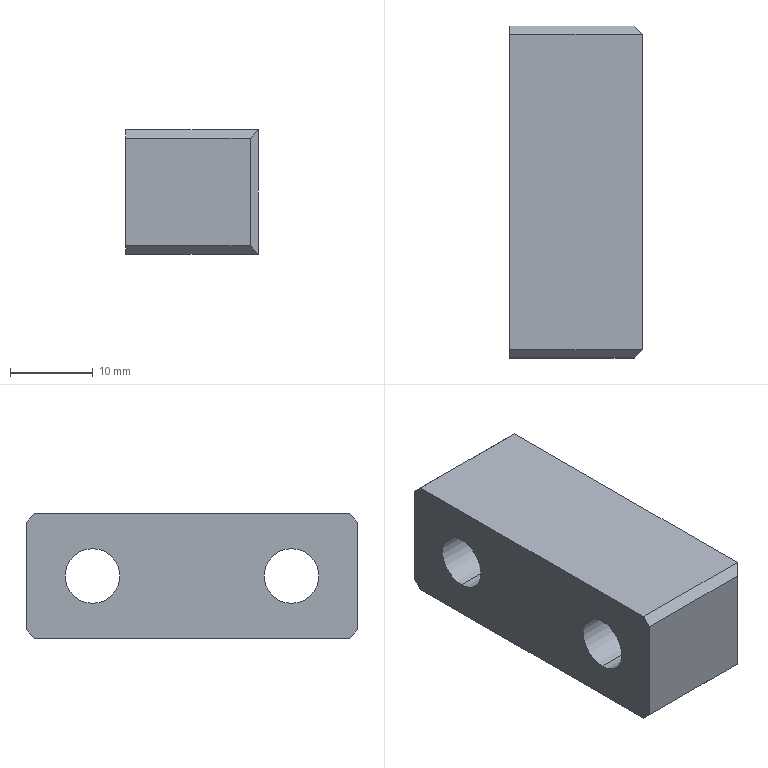Component | SolidWorks | ConveyorScrewAdjustmentSeatOne-2 | 1 solid | 22 faces | box 16 x 40 x 15 mm | volume 7389 mm3 | plane 14 | cylinder 8 | commonest cylinder face diameters 11 x4 6.6 x4 | material Plain Carbon Steel
build123d program:
from build123d import *

# Parameters (mm, degrees)
SKETCH1_W                                            = 15
SKETCH1_H                                            = 40
BOSS_EXTRUDE1_DEPTH                                  = 16
HOLE_SIZE_ACCORDING_TO_TYPE_1_OF_HEXAGON_D           = 6.6
HOLE_SIZE_ACCORDING_TO_TYPE_1_OF_HEXAGON_CBORE_D     = 11
HOLE_SIZE_ACCORDING_TO_TYPE_1_OF_HEXAGON_CBORE_DEPTH = 8.8
CHAMFER1_SIZE                                        = 1


with BuildPart() as part:
    # Sketch1 → Boss-Extrude1 (new body)
    with BuildSketch(Plane(origin=(0, 0, 0), x_dir=(0, 0, -1), z_dir=(1, 0, 0))):
        Rectangle(SKETCH1_W, SKETCH1_H)
    extrude(amount=BOSS_EXTRUDE1_DEPTH)

    # Hole Size according to type 1 of hexagon (through all)
    with Locations(Plane(origin=(16, 0, 0), x_dir=(0, 0, -1), z_dir=(1, 0, 0))):
        with Locations((0, 12), (0, -12)):
            CounterBoreHole(HOLE_SIZE_ACCORDING_TO_TYPE_1_OF_HEXAGON_D / 2, HOLE_SIZE_ACCORDING_TO_TYPE_1_OF_HEXAGON_CBORE_D / 2, HOLE_SIZE_ACCORDING_TO_TYPE_1_OF_HEXAGON_CBORE_DEPTH)

    # Chamfer1
    chamfer1_edges = [part.edges().sort_by_distance(p)[0] for p in [
        (16, -20, 0),
        (16, 20, 0),
        (8, -20, -7.5),
        (8, -20, 7.5),
        (8, 20, 7.5),
        (8, 20, -7.5),
    ]]
    chamfer(chamfer1_edges, length=CHAMFER1_SIZE)


solid = part.part

# Placed as in the assembly
solid = solid.moved(Location((47.45, 5.646, 227.5), (0, 0, 0)))
STEP:
#1=COLOUR_RGB('',0.7922,0.8196,0.9333);
#2=FILL_AREA_STYLE_COLOUR('',#1);
#3=FILL_AREA_STYLE('',(#2));
#4=SURFACE_STYLE_FILL_AREA(#3);
#5=SURFACE_SIDE_STYLE('',(#4));
#6=SURFACE_STYLE_USAGE(.BOTH.,#5);
#7=PRESENTATION_STYLE_ASSIGNMENT((#6));
#8=CARTESIAN_POINT('',(2.152,0.6947,9.173));
#9=VERTEX_POINT('',#8);
#10=CARTESIAN_POINT('',(2.152,0.6947,8.74));
#11=VERTEX_POINT('',#10);
#12=CARTESIAN_POINT('',(2.152,0.6947,8.957));
#13=DIRECTION('',(1.,0.,0.));
#14=DIRECTION('',(0.,0.,-1.));
#15=AXIS2_PLACEMENT_3D('',#12,#13,#14);
#16=CIRCLE('',#15,0.2165);
#17=EDGE_CURVE('',#9,#11,#16,.T.);
#18=ORIENTED_EDGE('',*,*,#17,.F.);
#19=CARTESIAN_POINT('',(2.498,0.6947,9.173));
#20=VERTEX_POINT('',#19);
#21=CARTESIAN_POINT('',(2.498,0.6947,9.173));
#22=DIRECTION('',(1.,0.,0.));
#23=VECTOR('',#22,39.37);
#24=LINE('',#21,#23);
#25=EDGE_CURVE('',#9,#20,#24,.T.);
#26=ORIENTED_EDGE('',*,*,#25,.T.);
#27=CARTESIAN_POINT('',(2.498,0.6947,8.74));
#28=VERTEX_POINT('',#27);
#29=CARTESIAN_POINT('',(2.498,0.6947,8.957));
#30=DIRECTION('',(1.,0.,0.));
#31=DIRECTION('',(0.,0.,-1.));
#32=AXIS2_PLACEMENT_3D('',#29,#30,#31);
#33=CIRCLE('',#32,0.2165);
#34=EDGE_CURVE('',#20,#28,#33,.T.);
#35=ORIENTED_EDGE('',*,*,#34,.T.);
#36=CARTESIAN_POINT('',(2.498,0.6947,8.74));
#37=DIRECTION('',(1.,0.,0.));
#38=VECTOR('',#37,39.37);
#39=LINE('',#36,#38);
#40=EDGE_CURVE('',#11,#28,#39,.T.);
#41=ORIENTED_EDGE('',*,*,#40,.F.);
#42=EDGE_LOOP('',(#18,#26,#35,#41));
#43=FACE_OUTER_BOUND('',#42,.T.);
#44=CARTESIAN_POINT('',(2.498,0.6947,8.957));
#45=DIRECTION('',(1.,0.,0.));
#46=DIRECTION('',(0.,0.,-1.));
#47=AXIS2_PLACEMENT_3D('',#44,#45,#46);
#48=CYLINDRICAL_SURFACE('',#47,0.2165);
#49=ADVANCED_FACE('',(#43),#48,.F.);
#50=CARTESIAN_POINT('',(1.868,0.6947,9.087));
#51=VERTEX_POINT('',#50);
#52=CARTESIAN_POINT('',(1.868,0.6947,8.827));
#53=VERTEX_POINT('',#52);
#54=CARTESIAN_POINT('',(1.868,0.6947,8.957));
#55=DIRECTION('',(1.,0.,0.));
#56=DIRECTION('',(0.,0.,-1.));
#57=AXIS2_PLACEMENT_3D('',#54,#55,#56);
#58=CIRCLE('',#57,0.1299);
#59=EDGE_CURVE('',#51,#53,#58,.T.);
#60=ORIENTED_EDGE('',*,*,#59,.F.);
#61=CARTESIAN_POINT('',(2.152,0.6947,9.087));
#62=VERTEX_POINT('',#61);
#63=CARTESIAN_POINT('',(2.498,0.6947,9.087));
#64=DIRECTION('',(1.,0.,0.));
#65=VECTOR('',#64,39.37);
#66=LINE('',#63,#65);
#67=EDGE_CURVE('',#51,#62,#66,.T.);
#68=ORIENTED_EDGE('',*,*,#67,.T.);
#69=CARTESIAN_POINT('',(2.152,0.6947,8.827));
#70=VERTEX_POINT('',#69);
#71=CARTESIAN_POINT('',(2.152,0.6947,8.957));
#72=DIRECTION('',(1.,0.,0.));
#73=DIRECTION('',(0.,0.,-1.));
#74=AXIS2_PLACEMENT_3D('',#71,#72,#73);
#75=CIRCLE('',#74,0.1299);
#76=EDGE_CURVE('',#62,#70,#75,.T.);
#77=ORIENTED_EDGE('',*,*,#76,.T.);
#78=CARTESIAN_POINT('',(2.498,0.6947,8.827));
#79=DIRECTION('',(1.,0.,0.));
#80=VECTOR('',#79,39.37);
#81=LINE('',#78,#80);
#82=EDGE_CURVE('',#53,#70,#81,.T.);
#83=ORIENTED_EDGE('',*,*,#82,.F.);
#84=EDGE_LOOP('',(#60,#68,#77,#83));
#85=FACE_OUTER_BOUND('',#84,.T.);
#86=CARTESIAN_POINT('',(2.498,0.6947,8.957));
#87=DIRECTION('',(1.,0.,0.));
#88=DIRECTION('',(0.,0.,-1.));
#89=AXIS2_PLACEMENT_3D('',#86,#87,#88);
#90=CYLINDRICAL_SURFACE('',#89,0.1299);
#91=ADVANCED_FACE('',(#85),#90,.F.);
#92=CARTESIAN_POINT('',(2.152,-0.2502,9.173));
#93=VERTEX_POINT('',#92);
#94=CARTESIAN_POINT('',(2.152,-0.2502,8.74));
#95=VERTEX_POINT('',#94);
#96=CARTESIAN_POINT('',(2.152,-0.2502,8.957));
#97=DIRECTION('',(1.,0.,0.));
#98=DIRECTION('',(0.,0.,-1.));
#99=AXIS2_PLACEMENT_3D('',#96,#97,#98);
#100=CIRCLE('',#99,0.2165);
#101=EDGE_CURVE('',#93,#95,#100,.T.);
#102=ORIENTED_EDGE('',*,*,#101,.F.);
#103=CARTESIAN_POINT('',(2.498,-0.2502,9.173));
#104=VERTEX_POINT('',#103);
#105=CARTESIAN_POINT('',(2.498,-0.2502,9.173));
#106=DIRECTION('',(1.,0.,0.));
#107=VECTOR('',#106,39.37);
#108=LINE('',#105,#107);
#109=EDGE_CURVE('',#93,#104,#108,.T.);
#110=ORIENTED_EDGE('',*,*,#109,.T.);
#111=CARTESIAN_POINT('',(2.498,-0.2502,8.74));
#112=VERTEX_POINT('',#111);
#113=CARTESIAN_POINT('',(2.498,-0.2502,8.957));
#114=DIRECTION('',(1.,0.,0.));
#115=DIRECTION('',(0.,0.,-1.));
#116=AXIS2_PLACEMENT_3D('',#113,#114,#115);
#117=CIRCLE('',#116,0.2165);
#118=EDGE_CURVE('',#104,#112,#117,.T.);
#119=ORIENTED_EDGE('',*,*,#118,.T.);
#120=CARTESIAN_POINT('',(2.498,-0.2502,8.74));
#121=DIRECTION('',(1.,0.,0.));
#122=VECTOR('',#121,39.37);
#123=LINE('',#120,#122);
#124=EDGE_CURVE('',#95,#112,#123,.T.);
#125=ORIENTED_EDGE('',*,*,#124,.F.);
#126=EDGE_LOOP('',(#102,#110,#119,#125));
#127=FACE_OUTER_BOUND('',#126,.T.);
#128=CARTESIAN_POINT('',(2.498,-0.2502,8.957));
#129=DIRECTION('',(1.,0.,0.));
#130=DIRECTION('',(0.,0.,-1.));
#131=AXIS2_PLACEMENT_3D('',#128,#129,#130);
#132=CYLINDRICAL_SURFACE('',#131,0.2165);
#133=ADVANCED_FACE('',(#127),#132,.F.);
#134=CARTESIAN_POINT('',(1.868,-0.2502,9.087));
#135=VERTEX_POINT('',#134);
#136=CARTESIAN_POINT('',(1.868,-0.2502,8.827));
#137=VERTEX_POINT('',#136);
#138=CARTESIAN_POINT('',(1.868,-0.2502,8.957));
#139=DIRECTION('',(1.,0.,0.));
#140=DIRECTION('',(0.,0.,-1.));
#141=AXIS2_PLACEMENT_3D('',#138,#139,#140);
#142=CIRCLE('',#141,0.1299);
#143=EDGE_CURVE('',#135,#137,#142,.T.);
#144=ORIENTED_EDGE('',*,*,#143,.F.);
#145=CARTESIAN_POINT('',(2.152,-0.2502,9.087));
#146=VERTEX_POINT('',#145);
#147=CARTESIAN_POINT('',(2.498,-0.2502,9.087));
#148=DIRECTION('',(1.,0.,0.));
#149=VECTOR('',#148,39.37);
#150=LINE('',#147,#149);
#151=EDGE_CURVE('',#135,#146,#150,.T.);
#152=ORIENTED_EDGE('',*,*,#151,.T.);
#153=CARTESIAN_POINT('',(2.152,-0.2502,8.827));
#154=VERTEX_POINT('',#153);
#155=CARTESIAN_POINT('',(2.152,-0.2502,8.957));
#156=DIRECTION('',(1.,0.,0.));
#157=DIRECTION('',(0.,0.,-1.));
#158=AXIS2_PLACEMENT_3D('',#155,#156,#157);
#159=CIRCLE('',#158,0.1299);
#160=EDGE_CURVE('',#146,#154,#159,.T.);
#161=ORIENTED_EDGE('',*,*,#160,.T.);
#162=CARTESIAN_POINT('',(2.498,-0.2502,8.827));
#163=DIRECTION('',(1.,0.,0.));
#164=VECTOR('',#163,39.37);
#165=LINE('',#162,#164);
#166=EDGE_CURVE('',#137,#154,#165,.T.);
#167=ORIENTED_EDGE('',*,*,#166,.F.);
#168=EDGE_LOOP('',(#144,#152,#161,#167));
#169=FACE_OUTER_BOUND('',#168,.T.);
#170=CARTESIAN_POINT('',(2.498,-0.2502,8.957));
#171=DIRECTION('',(1.,0.,0.));
#172=DIRECTION('',(0.,0.,-1.));
#173=AXIS2_PLACEMENT_3D('',#170,#171,#172);
#174=CYLINDRICAL_SURFACE('',#173,0.1299);
#175=ADVANCED_FACE('',(#169),#174,.F.);
#176=CARTESIAN_POINT('',(2.498,-0.5258,8.661));
#177=VERTEX_POINT('',#176);
#178=CARTESIAN_POINT('',(2.498,0.9703,8.661));
#179=VERTEX_POINT('',#178);
#180=CARTESIAN_POINT('',(2.498,-0.5651,8.661));
#181=DIRECTION('',(0.,1.,0.));
#182=VECTOR('',#181,39.37);
#183=LINE('',#180,#182);
#184=EDGE_CURVE('',#177,#179,#183,.T.);
#185=ORIENTED_EDGE('',*,*,#184,.F.);
#186=CARTESIAN_POINT('',(1.868,-0.5258,8.661));
#187=VERTEX_POINT('',#186);
#188=CARTESIAN_POINT('',(2.498,-0.5258,8.661));
#189=DIRECTION('',(-1.,0.,0.));
#190=VECTOR('',#189,39.37);
#191=LINE('',#188,#190);
#192=EDGE_CURVE('',#177,#187,#191,.T.);
#193=ORIENTED_EDGE('',*,*,#192,.T.);
#194=CARTESIAN_POINT('',(1.868,0.9703,8.661));
#195=VERTEX_POINT('',#194);
#196=CARTESIAN_POINT('',(1.868,-0.5651,8.661));
#197=DIRECTION('',(0.,1.,0.));
#198=VECTOR('',#197,39.37);
#199=LINE('',#196,#198);
#200=EDGE_CURVE('',#187,#195,#199,.T.);
#201=ORIENTED_EDGE('',*,*,#200,.T.);
#202=CARTESIAN_POINT('',(2.498,0.9703,8.661));
#203=DIRECTION('',(1.,0.,0.));
#204=VECTOR('',#203,39.37);
#205=LINE('',#202,#204);
#206=EDGE_CURVE('',#195,#179,#205,.T.);
#207=ORIENTED_EDGE('',*,*,#206,.T.);
#208=EDGE_LOOP('',(#185,#193,#201,#207));
#209=FACE_OUTER_BOUND('',#208,.T.);
#210=CARTESIAN_POINT('',(2.498,-0.5651,8.661));
#211=DIRECTION('',(0.,0.,1.));
#212=DIRECTION('',(1.,0.,0.));
#213=AXIS2_PLACEMENT_3D('',#210,#211,#212);
#214=PLANE('',#213);
#215=ADVANCED_FACE('',(#209),#214,.F.);
#216=CARTESIAN_POINT('',(1.868,1.01,8.701));
#217=VERTEX_POINT('',#216);
#218=CARTESIAN_POINT('',(1.868,1.01,9.213));
#219=VERTEX_POINT('',#218);
#220=CARTESIAN_POINT('',(1.868,1.01,9.252));
#221=DIRECTION('',(0.,0.,1.));
#222=VECTOR('',#221,39.37);
#223=LINE('',#220,#222);
#224=EDGE_CURVE('',#217,#219,#223,.T.);
#225=ORIENTED_EDGE('',*,*,#224,.T.);
#226=CARTESIAN_POINT('',(2.459,1.01,9.213));
#227=VERTEX_POINT('',#226);
#228=CARTESIAN_POINT('',(2.498,1.01,9.213));
#229=DIRECTION('',(1.,0.,0.));
#230=VECTOR('',#229,39.37);
#231=LINE('',#228,#230);
#232=EDGE_CURVE('',#219,#227,#231,.T.);
#233=ORIENTED_EDGE('',*,*,#232,.T.);
#234=CARTESIAN_POINT('',(2.459,1.01,8.701));
#235=VERTEX_POINT('',#234);
#236=CARTESIAN_POINT('',(2.459,1.01,9.252));
#237=DIRECTION('',(0.,0.,-1.));
#238=VECTOR('',#237,39.37);
#239=LINE('',#236,#238);
#240=EDGE_CURVE('',#227,#235,#239,.T.);
#241=ORIENTED_EDGE('',*,*,#240,.T.);
#242=CARTESIAN_POINT('',(2.498,1.01,8.701));
#243=DIRECTION('',(-1.,0.,0.));
#244=VECTOR('',#243,39.37);
#245=LINE('',#242,#244);
#246=EDGE_CURVE('',#235,#217,#245,.T.);
#247=ORIENTED_EDGE('',*,*,#246,.T.);
#248=EDGE_LOOP('',(#225,#233,#241,#247));
#249=FACE_OUTER_BOUND('',#248,.T.);
#250=CARTESIAN_POINT('',(2.498,1.01,9.252));
#251=DIRECTION('',(0.,-1.,0.));
#252=DIRECTION('',(0.,0.,-1.));
#253=AXIS2_PLACEMENT_3D('',#250,#251,#252);
#254=PLANE('',#253);
#255=ADVANCED_FACE('',(#249),#254,.F.);
#256=CARTESIAN_POINT('',(1.868,0.9703,9.252));
#257=VERTEX_POINT('',#256);
#258=CARTESIAN_POINT('',(1.868,-0.5258,9.252));
#259=VERTEX_POINT('',#258);
#260=CARTESIAN_POINT('',(1.868,-0.5651,9.252));
#261=DIRECTION('',(0.,-1.,0.));
#262=VECTOR('',#261,39.37);
#263=LINE('',#260,#262);
#264=EDGE_CURVE('',#257,#259,#263,.T.);
#265=ORIENTED_EDGE('',*,*,#264,.T.);
#266=CARTESIAN_POINT('',(2.498,-0.5258,9.252));
#267=VERTEX_POINT('',#266);
#268=CARTESIAN_POINT('',(2.498,-0.5258,9.252));
#269=DIRECTION('',(1.,0.,0.));
#270=VECTOR('',#269,39.37);
#271=LINE('',#268,#270);
#272=EDGE_CURVE('',#259,#267,#271,.T.);
#273=ORIENTED_EDGE('',*,*,#272,.T.);
#274=CARTESIAN_POINT('',(2.498,0.9703,9.252));
#275=VERTEX_POINT('',#274);
#276=CARTESIAN_POINT('',(2.498,-0.5651,9.252));
#277=DIRECTION('',(0.,-1.,0.));
#278=VECTOR('',#277,39.37);
#279=LINE('',#276,#278);
#280=EDGE_CURVE('',#275,#267,#279,.T.);
#281=ORIENTED_EDGE('',*,*,#280,.F.);
#282=CARTESIAN_POINT('',(2.498,0.9703,9.252));
#283=DIRECTION('',(-1.,0.,0.));
#284=VECTOR('',#283,39.37);
#285=LINE('',#282,#284);
#286=EDGE_CURVE('',#275,#257,#285,.T.);
#287=ORIENTED_EDGE('',*,*,#286,.T.);
#288=EDGE_LOOP('',(#265,#273,#281,#287));
#289=FACE_OUTER_BOUND('',#288,.T.);
#290=CARTESIAN_POINT('',(2.498,-0.5651,9.252));
#291=DIRECTION('',(0.,0.,-1.));
#292=DIRECTION('',(-1.,0.,0.));
#293=AXIS2_PLACEMENT_3D('',#290,#291,#292);
#294=PLANE('',#293);
#295=ADVANCED_FACE('',(#289),#294,.F.);
#296=CARTESIAN_POINT('',(1.868,-0.5651,9.213));
#297=VERTEX_POINT('',#296);
#298=CARTESIAN_POINT('',(1.868,-0.5651,8.701));
#299=VERTEX_POINT('',#298);
#300=CARTESIAN_POINT('',(1.868,-0.5651,9.252));
#301=DIRECTION('',(0.,0.,-1.));
#302=VECTOR('',#301,39.37);
#303=LINE('',#300,#302);
#304=EDGE_CURVE('',#297,#299,#303,.T.);
#305=ORIENTED_EDGE('',*,*,#304,.T.);
#306=CARTESIAN_POINT('',(2.459,-0.5651,8.701));
#307=VERTEX_POINT('',#306);
#308=CARTESIAN_POINT('',(2.498,-0.5651,8.701));
#309=DIRECTION('',(1.,0.,0.));
#310=VECTOR('',#309,39.37);
#311=LINE('',#308,#310);
#312=EDGE_CURVE('',#299,#307,#311,.T.);
#313=ORIENTED_EDGE('',*,*,#312,.T.);
#314=CARTESIAN_POINT('',(2.459,-0.5651,9.213));
#315=VERTEX_POINT('',#314);
#316=CARTESIAN_POINT('',(2.459,-0.5651,9.252));
#317=DIRECTION('',(0.,0.,1.));
#318=VECTOR('',#317,39.37);
#319=LINE('',#316,#318);
#320=EDGE_CURVE('',#307,#315,#319,.T.);
#321=ORIENTED_EDGE('',*,*,#320,.T.);
#322=CARTESIAN_POINT('',(2.498,-0.5651,9.213));
#323=DIRECTION('',(-1.,0.,0.));
#324=VECTOR('',#323,39.37);
#325=LINE('',#322,#324);
#326=EDGE_CURVE('',#315,#297,#325,.T.);
#327=ORIENTED_EDGE('',*,*,#326,.T.);
#328=EDGE_LOOP('',(#305,#313,#321,#327));
#329=FACE_OUTER_BOUND('',#328,.T.);
#330=CARTESIAN_POINT('',(2.498,-0.5651,9.252));
#331=DIRECTION('',(0.,1.,0.));
#332=DIRECTION('',(0.,0.,1.));
#333=AXIS2_PLACEMENT_3D('',#330,#331,#332);
#334=PLANE('',#333);
#335=ADVANCED_FACE('',(#329),#334,.F.);
#336=CARTESIAN_POINT('',(2.498,0.6947,8.957));
#337=DIRECTION('',(1.,0.,0.));
#338=DIRECTION('',(0.,0.,-1.));
#339=AXIS2_PLACEMENT_3D('',#336,#337,#338);
#340=CIRCLE('',#339,0.2165);
#341=EDGE_CURVE('',#28,#20,#340,.T.);
#342=ORIENTED_EDGE('',*,*,#341,.F.);
#343=ORIENTED_EDGE('',*,*,#34,.F.);
#344=EDGE_LOOP('',(#342,#343));
#345=FACE_BOUND('',#344,.T.);
#346=CARTESIAN_POINT('',(2.498,-0.2502,8.957));
#347=DIRECTION('',(1.,0.,0.));
#348=DIRECTION('',(0.,0.,-1.));
#349=AXIS2_PLACEMENT_3D('',#346,#347,#348);
#350=CIRCLE('',#349,0.2165);
#351=EDGE_CURVE('',#112,#104,#350,.T.);
#352=ORIENTED_EDGE('',*,*,#351,.F.);
#353=ORIENTED_EDGE('',*,*,#118,.F.);
#354=EDGE_LOOP('',(#352,#353));
#355=FACE_BOUND('',#354,.T.);
#356=ORIENTED_EDGE('',*,*,#280,.T.);
#357=CARTESIAN_POINT('',(2.498,-0.5258,8.957));
#358=DIRECTION('',(0.,0.,-1.));
#359=VECTOR('',#358,39.37);
#360=LINE('',#357,#359);
#361=EDGE_CURVE('',#267,#177,#360,.T.);
#362=ORIENTED_EDGE('',*,*,#361,.T.);
#363=ORIENTED_EDGE('',*,*,#184,.T.);
#364=CARTESIAN_POINT('',(2.498,0.9703,8.957));
#365=DIRECTION('',(0.,0.,1.));
#366=VECTOR('',#365,39.37);
#367=LINE('',#364,#366);
#368=EDGE_CURVE('',#179,#275,#367,.T.);
#369=ORIENTED_EDGE('',*,*,#368,.T.);
#370=EDGE_LOOP('',(#356,#362,#363,#369));
#371=FACE_OUTER_BOUND('',#370,.T.);
#372=CARTESIAN_POINT('',(2.498,0.2223,8.957));
#373=DIRECTION('',(-1.,0.,0.));
#374=DIRECTION('',(0.,0.,1.));
#375=AXIS2_PLACEMENT_3D('',#372,#373,#374);
#376=PLANE('',#375);
#377=ADVANCED_FACE('',(#345,#355,#371),#376,.F.);
#378=CARTESIAN_POINT('',(1.868,0.6947,8.957));
#379=DIRECTION('',(1.,0.,0.));
#380=DIRECTION('',(0.,0.,-1.));
#381=AXIS2_PLACEMENT_3D('',#378,#379,#380);
#382=CIRCLE('',#381,0.1299);
#383=EDGE_CURVE('',#53,#51,#382,.T.);
#384=ORIENTED_EDGE('',*,*,#383,.T.);
#385=ORIENTED_EDGE('',*,*,#59,.T.);
#386=EDGE_LOOP('',(#384,#385));
#387=FACE_BOUND('',#386,.T.);
#388=CARTESIAN_POINT('',(1.868,-0.2502,8.957));
#389=DIRECTION('',(1.,0.,0.));
#390=DIRECTION('',(0.,0.,-1.));
#391=AXIS2_PLACEMENT_3D('',#388,#389,#390);
#392=CIRCLE('',#391,0.1299);
#393=EDGE_CURVE('',#137,#135,#392,.T.);
#394=ORIENTED_EDGE('',*,*,#393,.T.);
#395=ORIENTED_EDGE('',*,*,#143,.T.);
#396=EDGE_LOOP('',(#394,#395));
#397=FACE_BOUND('',#396,.T.);
#398=ORIENTED_EDGE('',*,*,#200,.F.);
#399=CARTESIAN_POINT('',(1.868,-0.2994,8.435));
#400=DIRECTION('',(0.,-0.7071,0.7071));
#401=VECTOR('',#400,39.37);
#402=LINE('',#399,#401);
#403=EDGE_CURVE('',#187,#299,#402,.T.);
#404=ORIENTED_EDGE('',*,*,#403,.T.);
#405=ORIENTED_EDGE('',*,*,#304,.F.);
#406=CARTESIAN_POINT('',(1.868,-0.2994,9.478));
#407=DIRECTION('',(0.,0.7071,0.7071));
#408=VECTOR('',#407,39.37);
#409=LINE('',#406,#408);
#410=EDGE_CURVE('',#297,#259,#409,.T.);
#411=ORIENTED_EDGE('',*,*,#410,.T.);
#412=ORIENTED_EDGE('',*,*,#264,.F.);
#413=CARTESIAN_POINT('',(1.868,0.7439,9.478));
#414=DIRECTION('',(0.,0.7071,-0.7071));
#415=VECTOR('',#414,39.37);
#416=LINE('',#413,#415);
#417=EDGE_CURVE('',#257,#219,#416,.T.);
#418=ORIENTED_EDGE('',*,*,#417,.T.);
#419=ORIENTED_EDGE('',*,*,#224,.F.);
#420=CARTESIAN_POINT('',(1.868,0.7439,8.435));
#421=DIRECTION('',(0.,-0.7071,-0.7071));
#422=VECTOR('',#421,39.37);
#423=LINE('',#420,#422);
#424=EDGE_CURVE('',#217,#195,#423,.T.);
#425=ORIENTED_EDGE('',*,*,#424,.T.);
#426=EDGE_LOOP('',(#398,#404,#405,#411,#412,#418,#419,#425));
#427=FACE_OUTER_BOUND('',#426,.T.);
#428=CARTESIAN_POINT('',(1.868,0.2223,8.957));
#429=DIRECTION('',(-1.,0.,0.));
#430=DIRECTION('',(0.,0.,1.));
#431=AXIS2_PLACEMENT_3D('',#428,#429,#430);
#432=PLANE('',#431);
#433=ADVANCED_FACE('',(#387,#397,#427),#432,.T.);
#434=ORIENTED_EDGE('',*,*,#151,.F.);
#435=ORIENTED_EDGE('',*,*,#393,.F.);
#436=ORIENTED_EDGE('',*,*,#166,.T.);
#437=CARTESIAN_POINT('',(2.152,-0.2502,8.957));
#438=DIRECTION('',(1.,0.,0.));
#439=DIRECTION('',(0.,0.,-1.));
#440=AXIS2_PLACEMENT_3D('',#437,#438,#439);
#441=CIRCLE('',#440,0.1299);
#442=EDGE_CURVE('',#154,#146,#441,.T.);
#443=ORIENTED_EDGE('',*,*,#442,.T.);
#444=EDGE_LOOP('',(#434,#435,#436,#443));
#445=FACE_OUTER_BOUND('',#444,.T.);
#446=CARTESIAN_POINT('',(2.498,-0.2502,8.957));
#447=DIRECTION('',(1.,0.,0.));
#448=DIRECTION('',(0.,0.,-1.));
#449=AXIS2_PLACEMENT_3D('',#446,#447,#448);
#450=CYLINDRICAL_SURFACE('',#449,0.1299);
#451=ADVANCED_FACE('',(#445),#450,.F.);
#452=ORIENTED_EDGE('',*,*,#442,.F.);
#453=ORIENTED_EDGE('',*,*,#160,.F.);
#454=EDGE_LOOP('',(#452,#453));
#455=FACE_BOUND('',#454,.T.);
#456=CARTESIAN_POINT('',(2.152,-0.2502,8.957));
#457=DIRECTION('',(1.,0.,0.));
#458=DIRECTION('',(0.,0.,-1.));
#459=AXIS2_PLACEMENT_3D('',#456,#457,#458);
#460=CIRCLE('',#459,0.2165);
#461=EDGE_CURVE('',#95,#93,#460,.T.);
#462=ORIENTED_EDGE('',*,*,#461,.T.);
#463=ORIENTED_EDGE('',*,*,#101,.T.);
#464=EDGE_LOOP('',(#462,#463));
#465=FACE_OUTER_BOUND('',#464,.T.);
#466=CARTESIAN_POINT('',(2.152,-0.1202,8.957));
#467=DIRECTION('',(-1.,0.,0.));
#468=DIRECTION('',(0.,0.,1.));
#469=AXIS2_PLACEMENT_3D('',#466,#467,#468);
#470=PLANE('',#469);
#471=ADVANCED_FACE('',(#455,#465),#470,.F.);
#472=ORIENTED_EDGE('',*,*,#109,.F.);
#473=ORIENTED_EDGE('',*,*,#461,.F.);
#474=ORIENTED_EDGE('',*,*,#124,.T.);
#475=ORIENTED_EDGE('',*,*,#351,.T.);
#476=EDGE_LOOP('',(#472,#473,#474,#475));
#477=FACE_OUTER_BOUND('',#476,.T.);
#478=CARTESIAN_POINT('',(2.498,-0.2502,8.957));
#479=DIRECTION('',(1.,0.,0.));
#480=DIRECTION('',(0.,0.,-1.));
#481=AXIS2_PLACEMENT_3D('',#478,#479,#480);
#482=CYLINDRICAL_SURFACE('',#481,0.2165);
#483=ADVANCED_FACE('',(#477),#482,.F.);
#484=ORIENTED_EDGE('',*,*,#67,.F.);
#485=ORIENTED_EDGE('',*,*,#383,.F.);
#486=ORIENTED_EDGE('',*,*,#82,.T.);
#487=CARTESIAN_POINT('',(2.152,0.6947,8.957));
#488=DIRECTION('',(1.,0.,0.));
#489=DIRECTION('',(0.,0.,-1.));
#490=AXIS2_PLACEMENT_3D('',#487,#488,#489);
#491=CIRCLE('',#490,0.1299);
#492=EDGE_CURVE('',#70,#62,#491,.T.);
#493=ORIENTED_EDGE('',*,*,#492,.T.);
#494=EDGE_LOOP('',(#484,#485,#486,#493));
#495=FACE_OUTER_BOUND('',#494,.T.);
#496=CARTESIAN_POINT('',(2.498,0.6947,8.957));
#497=DIRECTION('',(1.,0.,0.));
#498=DIRECTION('',(0.,0.,-1.));
#499=AXIS2_PLACEMENT_3D('',#496,#497,#498);
#500=CYLINDRICAL_SURFACE('',#499,0.1299);
#501=ADVANCED_FACE('',(#495),#500,.F.);
#502=ORIENTED_EDGE('',*,*,#492,.F.);
#503=ORIENTED_EDGE('',*,*,#76,.F.);
#504=EDGE_LOOP('',(#502,#503));
#505=FACE_BOUND('',#504,.T.);
#506=CARTESIAN_POINT('',(2.152,0.6947,8.957));
#507=DIRECTION('',(1.,0.,0.));
#508=DIRECTION('',(0.,0.,-1.));
#509=AXIS2_PLACEMENT_3D('',#506,#507,#508);
#510=CIRCLE('',#509,0.2165);
#511=EDGE_CURVE('',#11,#9,#510,.T.);
#512=ORIENTED_EDGE('',*,*,#511,.T.);
#513=ORIENTED_EDGE('',*,*,#17,.T.);
#514=EDGE_LOOP('',(#512,#513));
#515=FACE_OUTER_BOUND('',#514,.T.);
#516=CARTESIAN_POINT('',(2.152,0.8246,8.957));
#517=DIRECTION('',(-1.,0.,0.));
#518=DIRECTION('',(0.,0.,1.));
#519=AXIS2_PLACEMENT_3D('',#516,#517,#518);
#520=PLANE('',#519);
#521=ADVANCED_FACE('',(#505,#515),#520,.F.);
#522=ORIENTED_EDGE('',*,*,#25,.F.);
#523=ORIENTED_EDGE('',*,*,#511,.F.);
#524=ORIENTED_EDGE('',*,*,#40,.T.);
#525=ORIENTED_EDGE('',*,*,#341,.T.);
#526=EDGE_LOOP('',(#522,#523,#524,#525));
#527=FACE_OUTER_BOUND('',#526,.T.);
#528=CARTESIAN_POINT('',(2.498,0.6947,8.957));
#529=DIRECTION('',(1.,0.,0.));
#530=DIRECTION('',(0.,0.,-1.));
#531=AXIS2_PLACEMENT_3D('',#528,#529,#530);
#532=CYLINDRICAL_SURFACE('',#531,0.2165);
#533=ADVANCED_FACE('',(#527),#532,.F.);
#534=ORIENTED_EDGE('',*,*,#410,.F.);
#535=ORIENTED_EDGE('',*,*,#326,.F.);
#536=CARTESIAN_POINT('',(2.4,-0.6242,9.154));
#537=DIRECTION('',(-0.5774,-0.5774,-0.5774));
#538=VECTOR('',#537,39.37);
#539=LINE('',#536,#538);
#540=EDGE_CURVE('',#267,#315,#539,.T.);
#541=ORIENTED_EDGE('',*,*,#540,.F.);
#542=ORIENTED_EDGE('',*,*,#272,.F.);
#543=EDGE_LOOP('',(#534,#535,#541,#542));
#544=FACE_OUTER_BOUND('',#543,.T.);
#545=CARTESIAN_POINT('',(2.498,-0.5651,9.213));
#546=DIRECTION('',(0.,0.7071,-0.7071));
#547=DIRECTION('',(-1.,0.,0.));
#548=AXIS2_PLACEMENT_3D('',#545,#546,#547);
#549=PLANE('',#548);
#550=ADVANCED_FACE('',(#544),#549,.F.);
#551=ORIENTED_EDGE('',*,*,#540,.T.);
#552=ORIENTED_EDGE('',*,*,#320,.F.);
#553=CARTESIAN_POINT('',(2.4,-0.6242,8.76));
#554=DIRECTION('',(-0.5774,-0.5774,0.5774));
#555=VECTOR('',#554,39.37);
#556=LINE('',#553,#555);
#557=EDGE_CURVE('',#177,#307,#556,.T.);
#558=ORIENTED_EDGE('',*,*,#557,.F.);
#559=ORIENTED_EDGE('',*,*,#361,.F.);
#560=EDGE_LOOP('',(#551,#552,#558,#559));
#561=FACE_OUTER_BOUND('',#560,.T.);
#562=CARTESIAN_POINT('',(2.498,-0.5258,8.957));
#563=DIRECTION('',(-0.7071,0.7071,0.));
#564=DIRECTION('',(0.,0.,-1.));
#565=AXIS2_PLACEMENT_3D('',#562,#563,#564);
#566=PLANE('',#565);
#567=ADVANCED_FACE('',(#561),#566,.F.);
#568=ORIENTED_EDGE('',*,*,#557,.T.);
#569=ORIENTED_EDGE('',*,*,#312,.F.);
#570=ORIENTED_EDGE('',*,*,#403,.F.);
#571=ORIENTED_EDGE('',*,*,#192,.F.);
#572=EDGE_LOOP('',(#568,#569,#570,#571));
#573=FACE_OUTER_BOUND('',#572,.T.);
#574=CARTESIAN_POINT('',(2.498,-0.5258,8.661));
#575=DIRECTION('',(0.,0.7071,0.7071));
#576=DIRECTION('',(-1.,0.,0.));
#577=AXIS2_PLACEMENT_3D('',#574,#575,#576);
#578=PLANE('',#577);
#579=ADVANCED_FACE('',(#573),#578,.F.);
#580=ORIENTED_EDGE('',*,*,#424,.F.);
#581=ORIENTED_EDGE('',*,*,#246,.F.);
#582=CARTESIAN_POINT('',(2.4,1.069,8.76));
#583=DIRECTION('',(-0.5774,0.5774,0.5774));
#584=VECTOR('',#583,39.37);
#585=LINE('',#582,#584);
#586=EDGE_CURVE('',#179,#235,#585,.T.);
#587=ORIENTED_EDGE('',*,*,#586,.F.);
#588=ORIENTED_EDGE('',*,*,#206,.F.);
#589=EDGE_LOOP('',(#580,#581,#587,#588));
#590=FACE_OUTER_BOUND('',#589,.T.);
#591=CARTESIAN_POINT('',(2.498,1.01,8.701));
#592=DIRECTION('',(0.,-0.7071,0.7071));
#593=DIRECTION('',(-1.,0.,0.));
#594=AXIS2_PLACEMENT_3D('',#591,#592,#593);
#595=PLANE('',#594);
#596=ADVANCED_FACE('',(#590),#595,.F.);
#597=ORIENTED_EDGE('',*,*,#586,.T.);
#598=ORIENTED_EDGE('',*,*,#240,.F.);
#599=CARTESIAN_POINT('',(2.4,1.069,9.154));
#600=DIRECTION('',(-0.5774,0.5774,-0.5774));
#601=VECTOR('',#600,39.37);
#602=LINE('',#599,#601);
#603=EDGE_CURVE('',#275,#227,#602,.T.);
#604=ORIENTED_EDGE('',*,*,#603,.F.);
#605=ORIENTED_EDGE('',*,*,#368,.F.);
#606=EDGE_LOOP('',(#597,#598,#604,#605));
#607=FACE_OUTER_BOUND('',#606,.T.);
#608=CARTESIAN_POINT('',(2.498,0.9703,8.957));
#609=DIRECTION('',(-0.7071,-0.7071,0.));
#610=DIRECTION('',(0.,0.,1.));
#611=AXIS2_PLACEMENT_3D('',#608,#609,#610);
#612=PLANE('',#611);
#613=ADVANCED_FACE('',(#607),#612,.F.);
#614=ORIENTED_EDGE('',*,*,#603,.T.);
#615=ORIENTED_EDGE('',*,*,#232,.F.);
#616=ORIENTED_EDGE('',*,*,#417,.F.);
#617=ORIENTED_EDGE('',*,*,#286,.F.);
#618=EDGE_LOOP('',(#614,#615,#616,#617));
#619=FACE_OUTER_BOUND('',#618,.T.);
#620=CARTESIAN_POINT('',(2.498,0.9703,9.252));
#621=DIRECTION('',(0.,-0.7071,-0.7071));
#622=DIRECTION('',(-1.,0.,0.));
#623=AXIS2_PLACEMENT_3D('',#620,#621,#622);
#624=PLANE('',#623);
#625=ADVANCED_FACE('',(#619),#624,.F.);
#626=CLOSED_SHELL('',(#49,#91,#133,#175,#215,#255,#295,#335,#377,#433,#451,#471,#483,#501,#521,#533,#550,#567,#579,#596,#613,#625));
#627=MANIFOLD_SOLID_BREP('',#626);
#628=STYLED_ITEM('',(#7),#627);
#629=(LENGTH_UNIT()NAMED_UNIT(*)SI_UNIT($,.METRE.));
#630=LENGTH_MEASURE_WITH_UNIT(LENGTH_MEASURE(0.0254),#629);
#631=DIMENSIONAL_EXPONENTS(1.,0.,0.,0.,0.,0.,0.);
#632=(CONVERSION_BASED_UNIT('',#630)LENGTH_UNIT()NAMED_UNIT(#631));
#633=UNCERTAINTY_MEASURE_WITH_UNIT(LENGTH_MEASURE(0.00001),#632,'','');
#634=(NAMED_UNIT(*)PLANE_ANGLE_UNIT()SI_UNIT($,.RADIAN.));
#635=(NAMED_UNIT(*)SI_UNIT($,.STERADIAN.)SOLID_ANGLE_UNIT());
#636=(GEOMETRIC_REPRESENTATION_CONTEXT(3)GLOBAL_UNCERTAINTY_ASSIGNED_CONTEXT((#633))GLOBAL_UNIT_ASSIGNED_CONTEXT((#632,#634,#635))REPRESENTATION_CONTEXT('',''));
#637=MECHANICAL_DESIGN_GEOMETRIC_PRESENTATION_REPRESENTATION('',(#628),#636);
#638=CARTESIAN_POINT('',(0.,0.,0.));
#639=DIRECTION('',(0.,0.,1.));
#640=DIRECTION('',(1.,0.,0.));
#641=AXIS2_PLACEMENT_3D('',#638,#639,#640);
#642=(LENGTH_UNIT()NAMED_UNIT(*)SI_UNIT($,.METRE.));
#643=LENGTH_MEASURE_WITH_UNIT(LENGTH_MEASURE(0.0254),#642);
#644=DIMENSIONAL_EXPONENTS(1.,0.,0.,0.,0.,0.,0.);
#645=(CONVERSION_BASED_UNIT('',#643)LENGTH_UNIT()NAMED_UNIT(#644));
#646=UNCERTAINTY_MEASURE_WITH_UNIT(LENGTH_MEASURE(0.00001),#645,'','');
#647=(NAMED_UNIT(*)PLANE_ANGLE_UNIT()SI_UNIT($,.RADIAN.));
#648=(NAMED_UNIT(*)SI_UNIT($,.STERADIAN.)SOLID_ANGLE_UNIT());
#649=(GEOMETRIC_REPRESENTATION_CONTEXT(3)GLOBAL_UNCERTAINTY_ASSIGNED_CONTEXT((#646))GLOBAL_UNIT_ASSIGNED_CONTEXT((#645,#647,#648))REPRESENTATION_CONTEXT('',''));
#650=ADVANCED_BREP_SHAPE_REPRESENTATION('',(#627,#641),#649);
#651=PRESENTATION_LAYER_ASSIGNMENT('','',(#628));